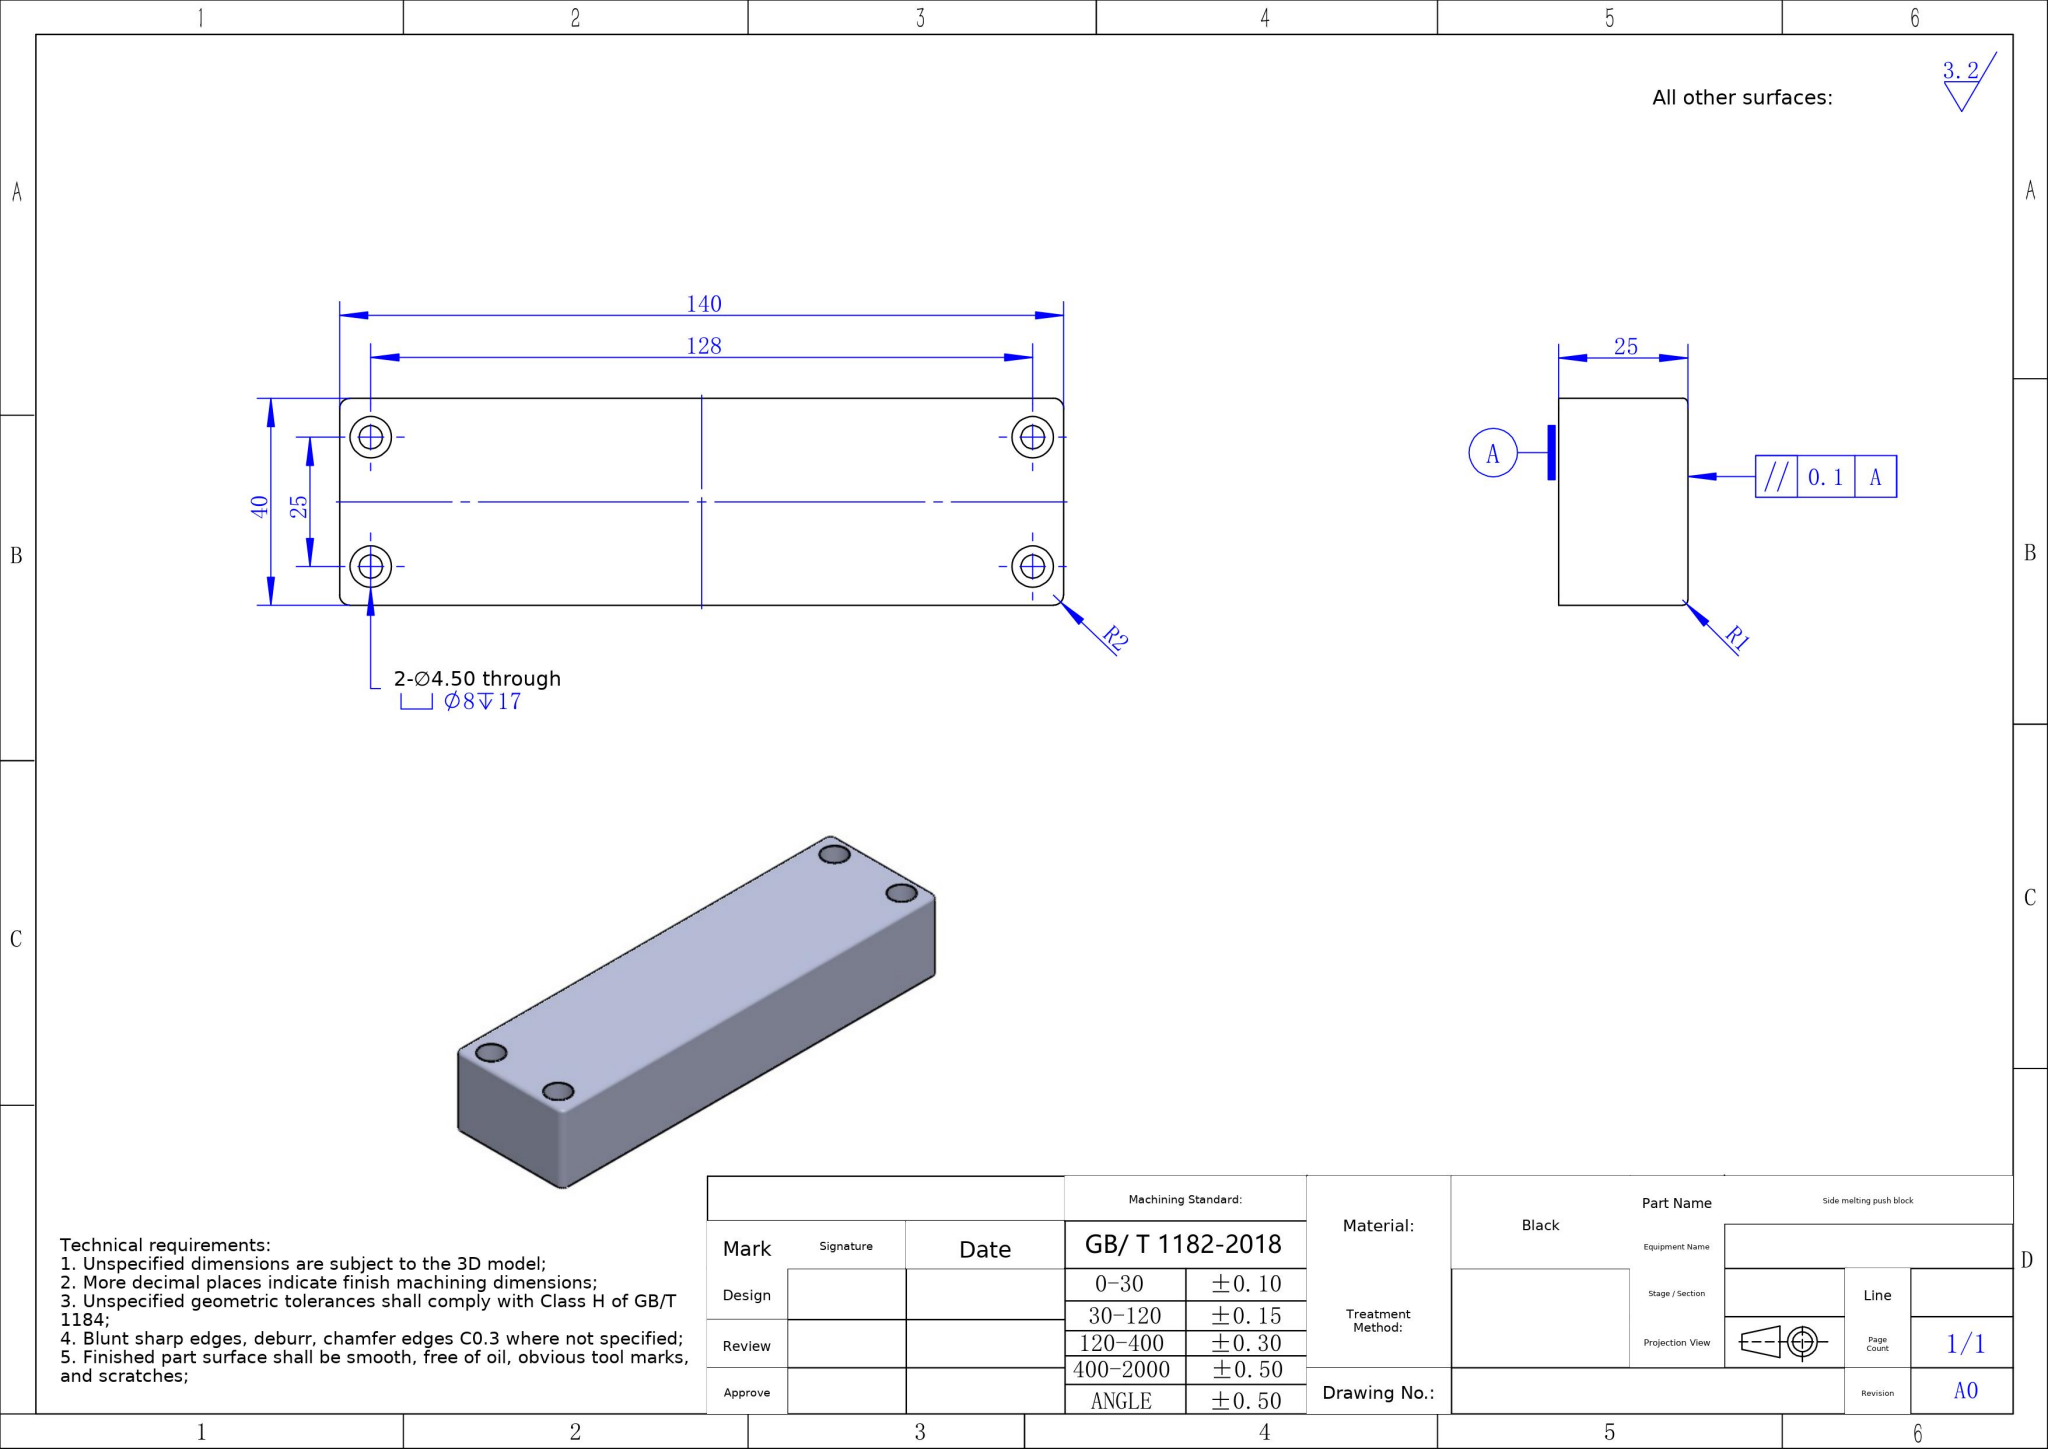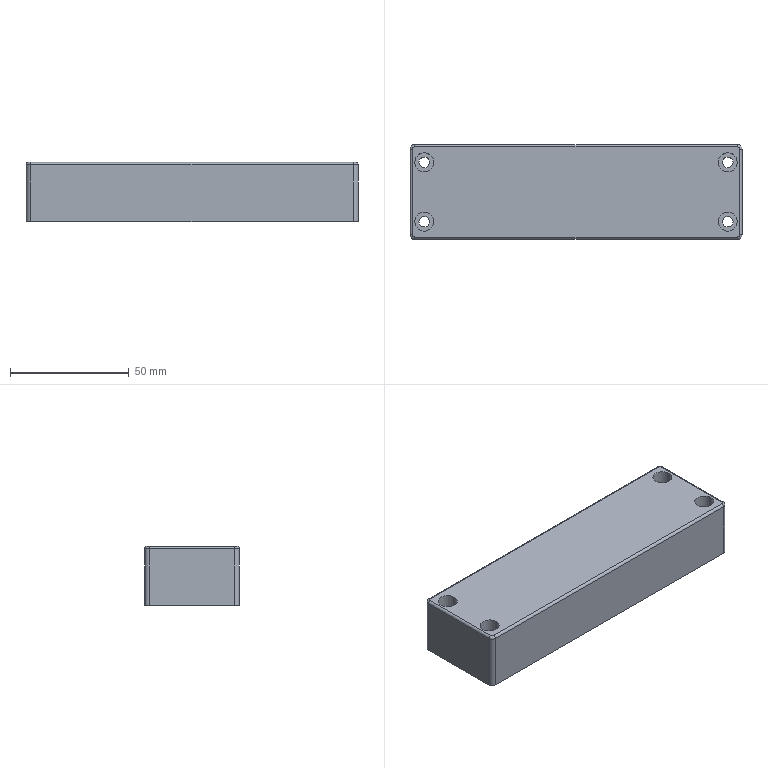Part | SolidWorks | mm | material Black | 1 solid | 38 faces | box 140 x 40 x 25 mm | volume 135911 mm3 | cylinder 24 | plane 10 | torus 4 | commonest cylinder face diameters 8 x8 4.5 x8 4 x4 2 x4
build123d program:
from build123d import *

# Parameters (mm, degrees)
SKETCH1_W                                          = 140
SKETCH1_H                                          = 40
BOSS_EXTRUDE1_DEPTH                                = 25
HOLE_SIZE_ACCORDING_TO_TYPE_2_OF_HEXAG_D           = 4.5
HOLE_SIZE_ACCORDING_TO_TYPE_2_OF_HEXAG_CBORE_D     = 8
HOLE_SIZE_ACCORDING_TO_TYPE_2_OF_HEXAG_CBORE_DEPTH = 17
FILLET1_R                                          = 2
FILLET2_R                                          = 1


with BuildPart() as part:
    # Sketch1 → Boss-Extrude1 (new body)
    with BuildSketch(Plane.XY):
        Rectangle(SKETCH1_W, SKETCH1_H)
    extrude(amount=BOSS_EXTRUDE1_DEPTH)

    # Hole Size _According to_ Type 2 of Hexag (through all)
    with Locations(Plane.XY.offset(25)):
        with Locations((-64, 12.5), (64, 12.5), (64, -12.5), (-64, -12.5)):
            CounterBoreHole(HOLE_SIZE_ACCORDING_TO_TYPE_2_OF_HEXAG_D / 2, HOLE_SIZE_ACCORDING_TO_TYPE_2_OF_HEXAG_CBORE_D / 2, HOLE_SIZE_ACCORDING_TO_TYPE_2_OF_HEXAG_CBORE_DEPTH)

    # Fillet1
    fillet1_edges = [part.edges().sort_by_distance(p)[0] for p in [
        (70, -20, 12.5),
        (-70, -20, 12.5),
        (-70, 20, 12.5),
        (70, 20, 12.5),
    ]]
    fillet(fillet1_edges, radius=FILLET1_R)

    # Fillet2
    fillet2_edges = [part.edges().sort_by_distance(p)[0] for p in [
        (70, 0, 25),
        (0, -20, 25),
        (0, 20, 25),
        (-70, 0, 25),
        (-69.414, 19.414, 25),
        (69.414, 19.414, 25),
        (-69.414, -19.414, 25),
        (69.414, -19.414, 25),
    ]]
    fillet(fillet2_edges, radius=FILLET2_R)


solid = part.part